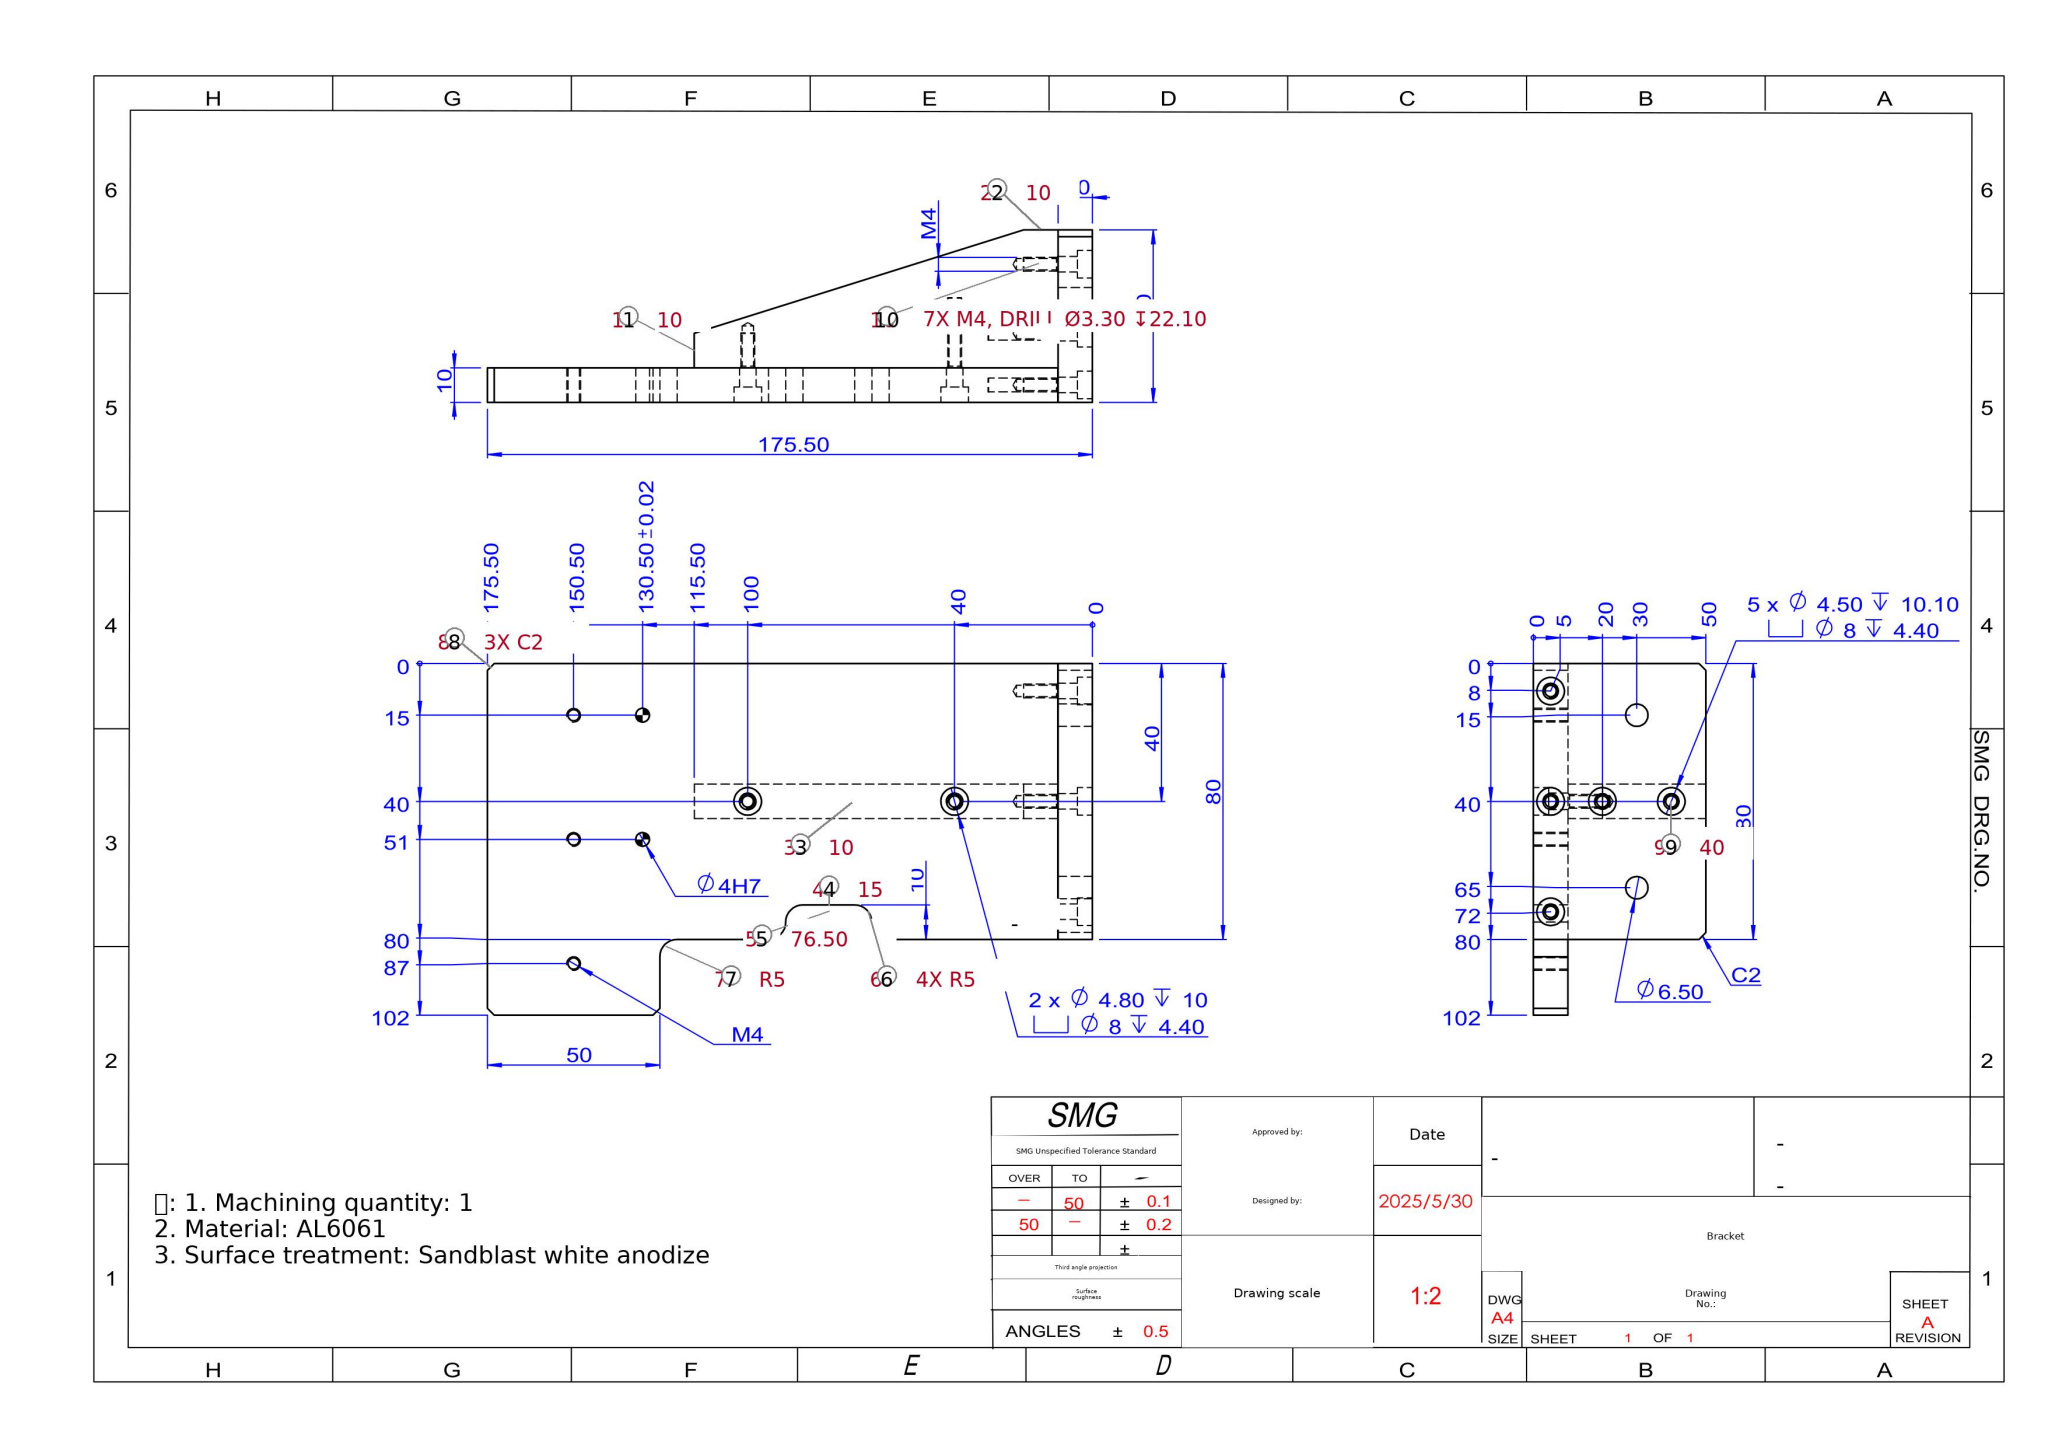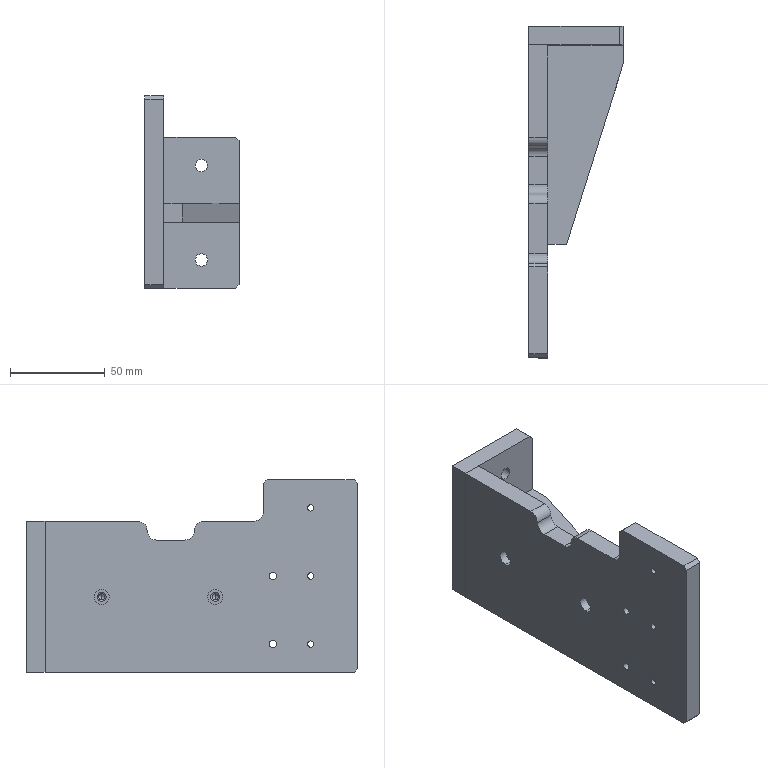Part | SolidWorks | mm | material AL6061 | 1 solid | 128 faces | box 50 x 175.5 x 102 mm | volume 204595 mm3 | cylinder 67 | plane 33 | cone 28 | commonest cylinder face diameters 3.3 x20 4.5 x16 8 x14 10 x5 4 x4 4.8 x4 6.5 x4